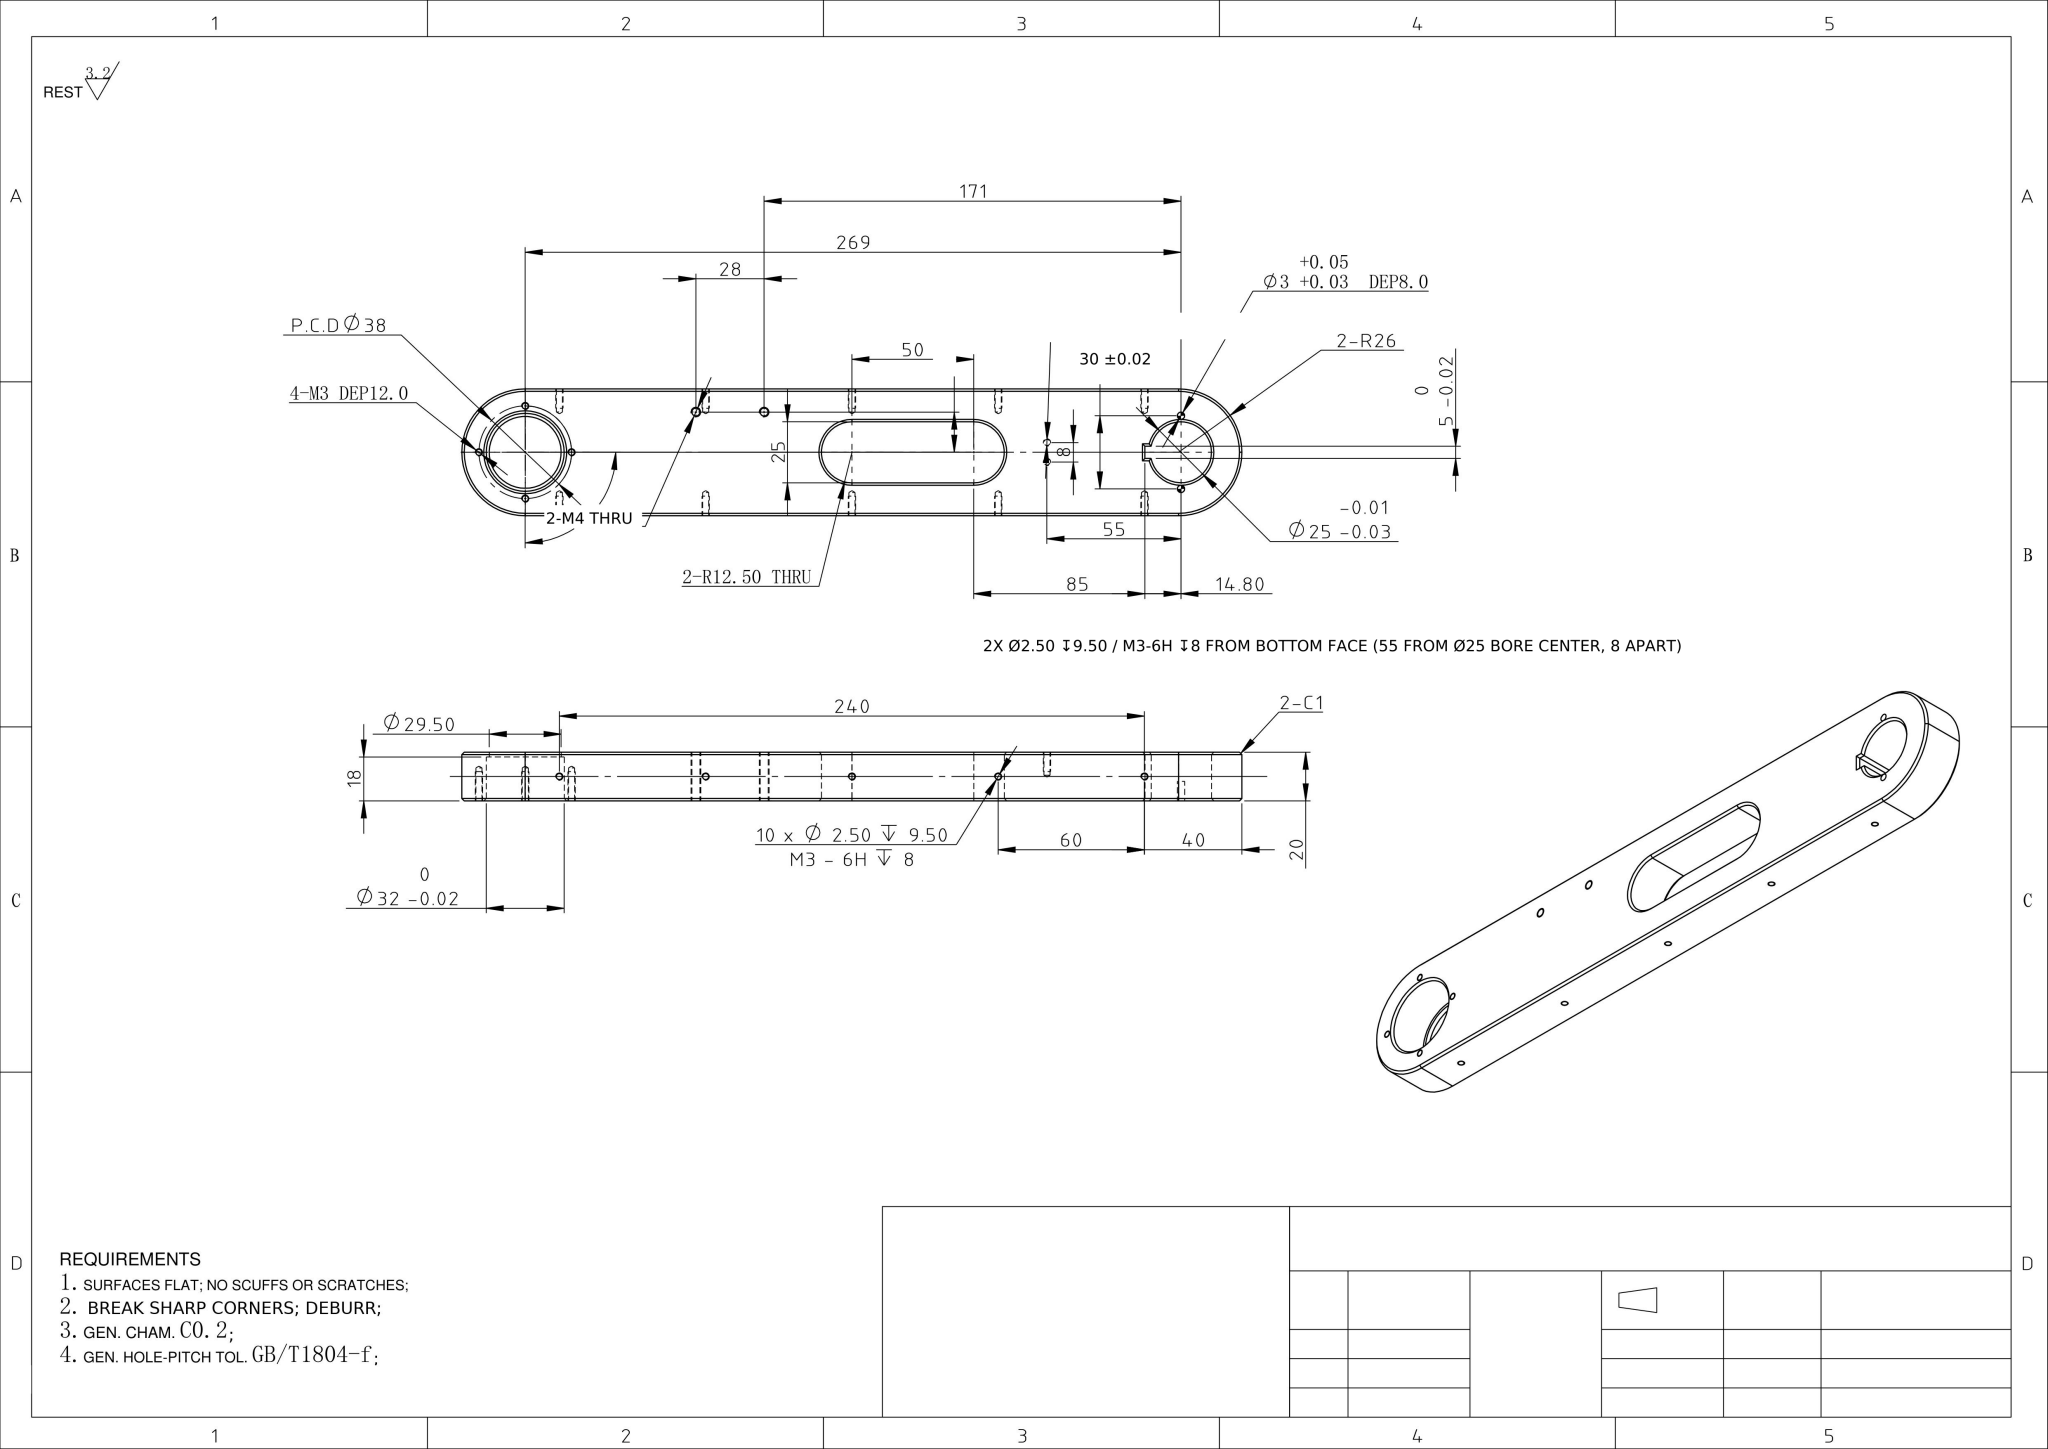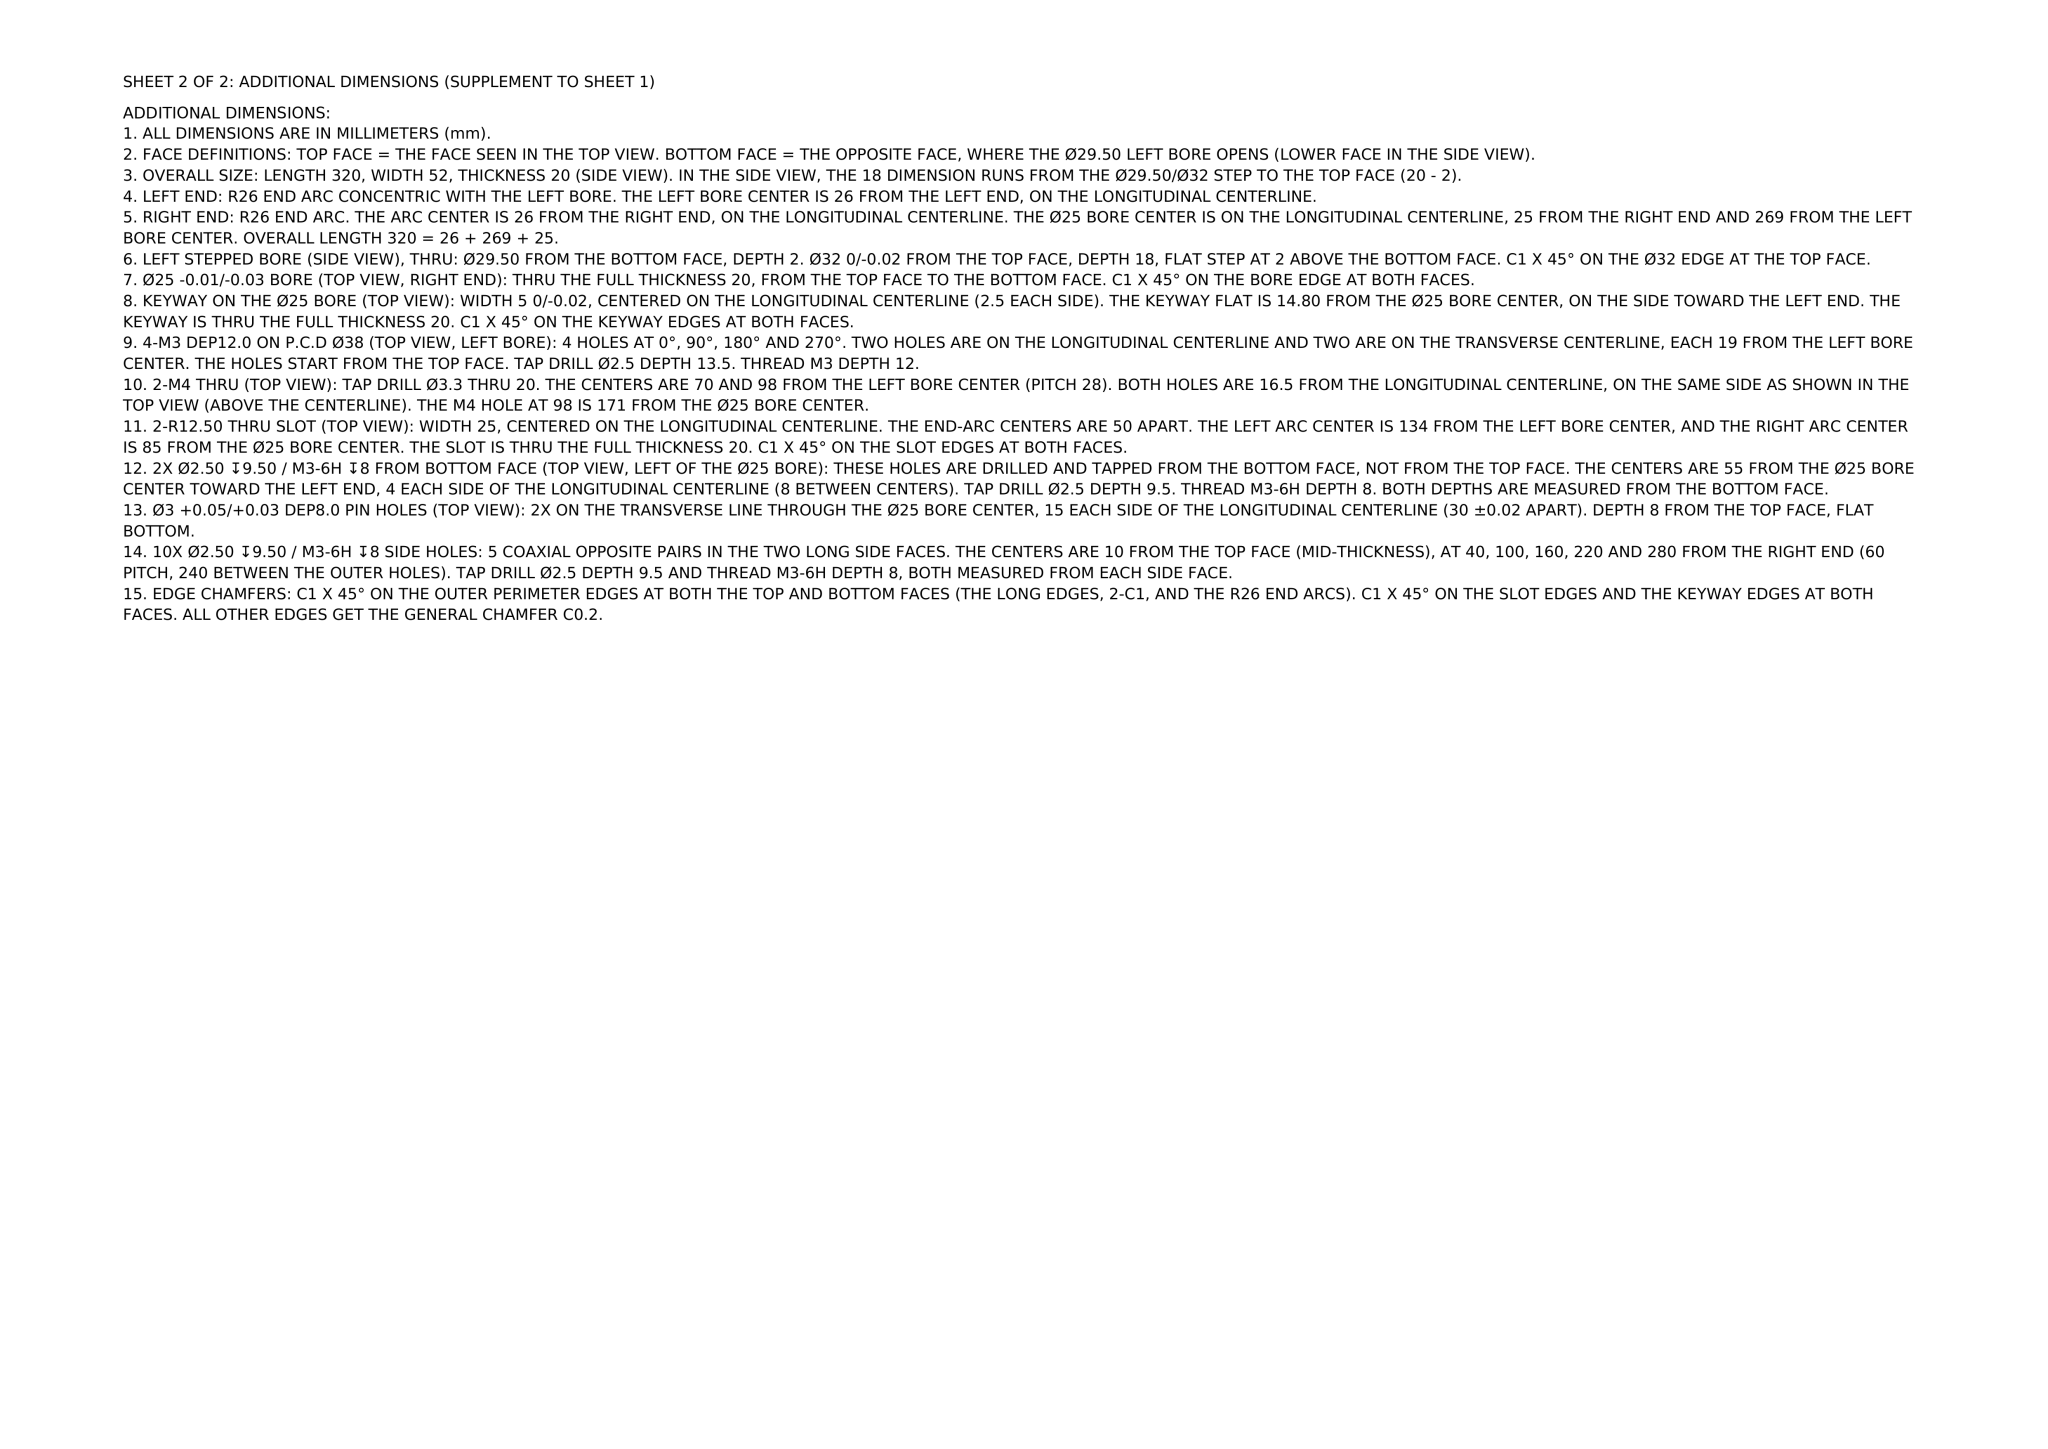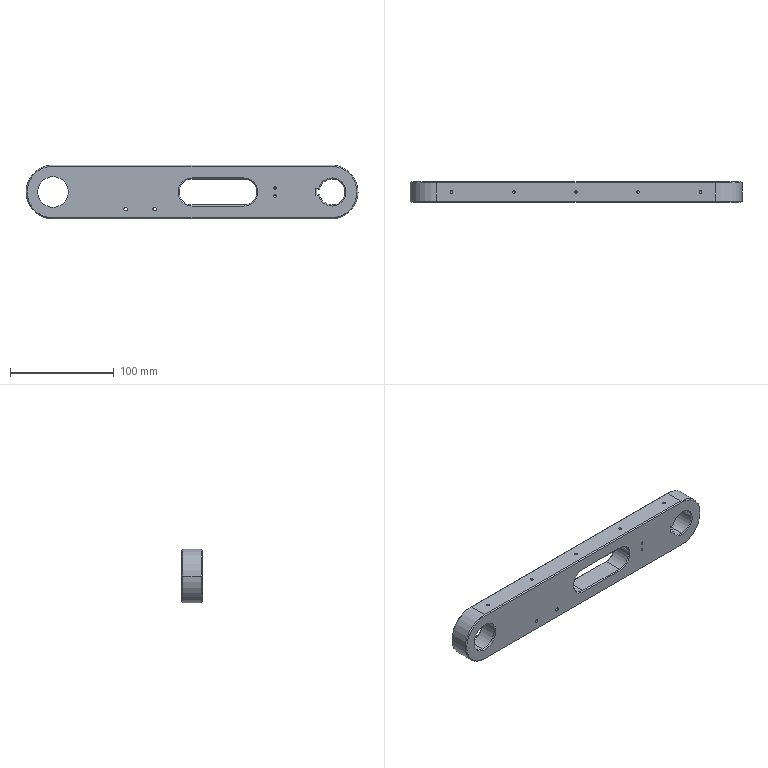Part | NX | mm | 1 solid | 131 faces | box 320 x 20 x 52 mm | volume 258163 mm3 | cylinder 53 | cone 52 | plane 26 | commonest cylinder face diameters 2.5 x32 25 x5 3 x4 3.3 x4 52 x4 29.5 x2 32 x2